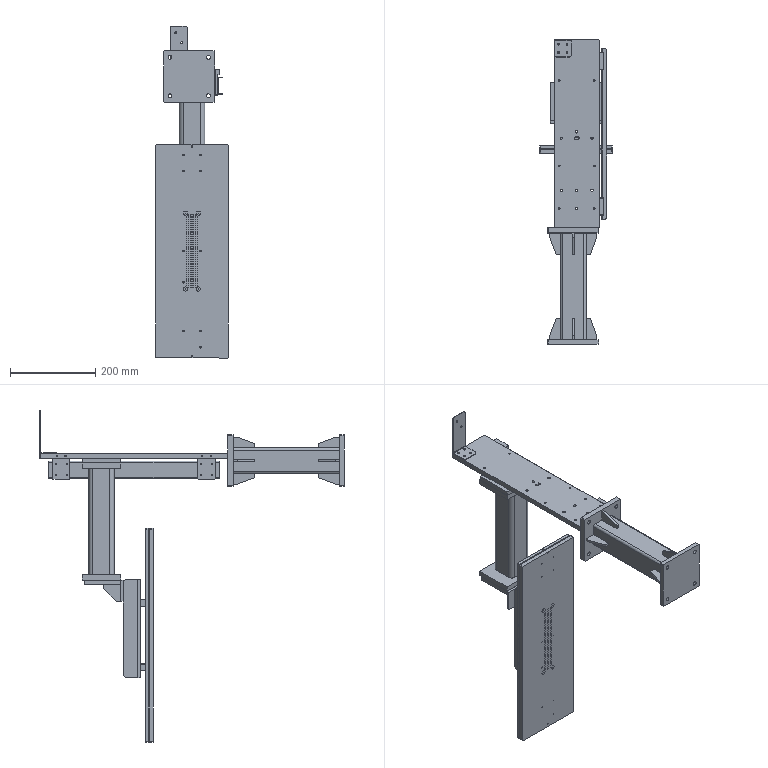Assembly | SolidWorks | mm | 18 component files | 28 solids | 1241 faces | box 170 x 712 x 777.07 mm | volume 4280144 mm3 | cylinder 823 | plane 322 | cone 96 | commonest cylinder face diameters 0.6 x482 3.3 x56 4.2 x44 4.5 x40 10 x40 5.5 x40 8 x24 2.5 x20
Bill of materials:
001 | 1 | Q235B | Welded-style frame made of a long channel or I-section member running between two square end plates, with triangular gusset ribs at both ends.
005 | 1 | AL6061 | Long, thin rectangular plate with a scattered pattern of small holes and one slot on the main face, plus small holes in the narrow edge faces.
006 | 1 | AL6061 | Thick rectangular plate with a grid of round through holes in several sizes and one obround slot.
007 | 1 | AL6061 | Plain solid rectangular plate or block with no visible holes or cutouts.
008 | 1 | AL6061 | Thin rectangular plate with two large round through holes, each flanked by two small holes, plus small holes along the long edges.
009 | 2 | AL6061 | Long rectangular bar with chamfered corners along one long edge at both ends and three small holes in one narrow face.
011 | 2 | AL6061 | Rectangular block with three large round through holes in a row through its main face.
012 | 1 | AL6061 | Thin rectangular sheet or panel with small holes along both long edges and larger holes on the centerline near each end.
013 | 1 | AL6061 | Thin rectangular sheet or panel with a faint dotted pattern in a narrow vertical region near the center of one face.
015 | 1 | SUS304 | Bent L-shaped bracket made of plate with rounded outer corners, holes in both legs.
017 | 1 | SUS304 | Long formed C-channel (U-profile) with rounded bends and groups of small holes near each end of the web.
021 | 1 | AL6061 | Plain thin rectangular plate with no visible holes.
022 | 1 | AL6061 | Solid block shaped like a corner gusset with a constant thickness. Its side profile has a full-width straight top edge, a full-height vertical back edge, a short vertical edge at the outer end, and a long diagonal edge running down to a narrow flat bottom. There are two round holes in the top face and two in the vertical back face.
023 | 1 |  | Column shaped like an I-beam: two flat rectangular end plates of the same size joined by a central rectangular post. The post is narrower than the plates and has rounded vertical edges.
X003.02-011(1)-014 | 2 | AL6061 | Rectangular plate with a thicker stepped lip along one edge, so its side profile is L-shaped. It has two larger round through-holes near the lip edge and four smaller round through-holes in a rectangular pattern lower on the plate. The plate corners are very slightly rounded or chamfered.
Mates:
1. parallel | 006-1 face at (-180.455, -15.942, 144.696) dir (0, 1, 0) | 007-1 face at (-180.455, -21.942, -139.304) dir (0, 1, 0)
2. concentric | 008-2 face at (-275.455, -151.942, -338.376) dir (0, -1, 0) r 2.75 | 009-2 face at (-275.455, -145.942, -338.376) dir (0, -1, 0) r 2.1
3. concentric | 008-2 face at (-275.455, -151.942, -243.376) dir (0, -1, 0) r 2.75 | 009-2 face at (-275.455, -145.942, -243.376) dir (0, -1, 0) r 2.1
4. coincident | 008-2 face at (-240.455, -145.942, -238.376) dir (0, 1, 0) | 009-2 face at (-270.455, -145.942, -358.376) dir (0, -1, 0)
5. concentric | 008-2 face at (-205.455, -151.942, -338.376) dir (0, -1, 0) r 2.75 | 009-1 face at (-205.455, -145.942, -338.376) dir (0, -1, 0) r 2.1
6. concentric | 008-2 face at (-205.455, -151.942, -243.376) dir (0, -1, 0) r 2.75 | 009-1 face at (-205.455, -145.942, -243.376) dir (0, -1, 0) r 2.1
7. coincident | 008-2 face at (-240.455, -145.942, -238.376) dir (0, 1, 0) | 009-1 face at (-200.455, -145.942, -358.376) dir (0, -1, 0)
8. concentric | 011-1 face at (-228.955, -151.942, -183.376) dir (0, 1, 0) r 5 | 012-1 face at (-228.955, -163.942, -183.376) dir (0, 1, 0) r 2.1
9. coincident | 011-1 face at (-240.455, -163.942, -183.376) dir (0, -1, 0) | 012-1 face at (-240.455, -163.942, -258.376) dir (0, 1, 0)
10. concentric | 011-1 face at (-251.955, -151.942, -183.376) dir (0, 1, 0) r 5 | 012-1 face at (-251.955, -163.942, -183.376) dir (0, 1, 0) r 2.1
11. coincident | 011-2 face at (-240.455, -163.942, -333.376) dir (0, -1, 0) | 012-1 face at (-240.455, -163.942, -258.376) dir (0, 1, 0)
12. concentric | 011-2 face at (-228.955, -151.942, -333.376) dir (0, 1, 0) r 5 | 012-1 face at (-228.955, -163.942, -333.376) dir (0, 1, 0) r 2.1
13. concentric | 011-2 face at (-251.955, -151.942, -333.376) dir (0, 1, 0) r 2.75 | 012-1 face at (-251.955, -163.942, -333.376) dir (0, 1, 0) r 2.1
14. coincident | 012-1 face at (-240.455, -171.942, -258.376) dir (0, -1, 0) | 013-1 face at (-240.455, -171.942, -258.376) dir (0, 1, 0)
15. coincident | 012-1 face at (-325.455, -171.942, -8.376) dir (-1, 0, 0) | 013-1 face at (-325.455, -181.942, -8.376) dir (-1, 0, 0)
16. coincident | 012-1 face at (-325.455, -171.942, -508.376) dir (0, 0, -1) | 013-1 face at (-325.455, -181.942, -508.376) dir (0, 0, -1)
17. coincident | X003.02-011(1)-014-2 face at (-186.455, -306.942, 136.696) dir (-1, 0, 0) | 005-1 face at (-186.455, -356.942, 154.696) dir (1, 0, 0)
18. concentric | X003.02-011(1)-014-2 face at (-186.455, -316.942, 160.696) dir (-1, 0, 0) r 2.25 | 005-1 face at (-186.455, -316.942, 160.696) dir (1, 0, 0) r 1.65
19. concentric | X003.02-011(1)-014-2 face at (-186.455, -296.942, 160.696) dir (-1, 0, 0) r 2.25 | 005-1 face at (-186.455, -296.942, 160.696) dir (1, 0, 0) r 1.65
20. coincident | 005-1 face at (-238.955, -136.942, 166.696) dir (0, 0, 1) | 015-1 face at (-271.455, 63.058, 166.696) dir (0, 0, -1)
21. concentric | 005-1 face at (-261.455, 53.058, 166.696) dir (0, 0, 1) r 1.65 | 015-1 face at (-261.455, 53.058, 166.696) dir (0, 0, 1) r 2.25
22. coincident | 005-1 face at (-186.455, 83.058, 154.696) dir (0, 1, 0) | 015-1 face at (-271.455, 83.058, 168.196) dir (0, 1, 0)
23. coincident | 021-1 face at (-240.455, -105.942, -154.304) dir (0, 1, 0) | 022-1 face at (-235.455, -105.942, -139.304) dir (0, -1, 0)
24. coincident | 009-2 face at (-270.455, -111.942, -128.376) dir (0, 1, 0) | 021-1 face at (-240.455, -111.942, -154.304) dir (0, -1, 0)
25. coincident | 006-1 face at (-240.455, -60.942, 144.696) dir (0, 0, -1) | 023-1 face at (-240.455, -60.942, 144.696) dir (0, 0, 1)
26. coincident | 006-1 face at (-180.455, -105.942, 144.696) dir (0, -1, 0) | 023-1 face at (-300.455, -105.942, 132.696) dir (0, -1, 0)
27. width | 023-1 face at (-300.455, -15.942, 132.696) dir (-1, 0, 0) | 023-1 face at (-180.455, -15.942, 132.696) dir (1, 0, 0) | 006-1 face at (-300.455, -105.942, 144.696) dir (-1, 0, 0) | 006-1 face at (-180.455, -105.942, 144.696) dir (1, 0, 0)
28. coincident | X003.02-011(1)-014-2 face at (-180.455, -306.942, 136.696) dir (1, 0, 0) | 017-1 face at (-180.455, -136.942, 129.196) dir (-1, 0, 0)
29. coincident | X003.02-011(1)-014-1 face at (-186.455, 33.058, 136.696) dir (-1, 0, 0) | 005-1 face at (-186.455, -356.942, 154.696) dir (1, 0, 0)
30. concentric | X003.02-011(1)-014-1 face at (-186.455, 43.058, 160.696) dir (-1, 0, 0) r 2.25 | 005-1 face at (-186.455, 43.058, 160.696) dir (1, 0, 0) r 1.65
31. concentric | X003.02-011(1)-014-1 face at (-186.455, 23.058, 160.696) dir (-1, 0, 0) r 2.25 | 005-1 face at (-186.455, 23.058, 160.696) dir (1, 0, 0) r 1.65
32. concentric | X003.02-011(1)-014-1 edge at (-180.455, 45.558, 141.696) dir (1, 0, 0) r 1.25 | 017-1 edge at (-178.955, 45.558, 141.696) dir (1, 0, 0) r 3.3
33. concentric | X003.02-011(1)-014-2 edge at (-180.455, -319.442, 141.696) dir (1, 0, 0) r 1.25 | 017-1 edge at (-178.955, -319.442, 141.696) dir (1, 0, 0) r 3.3
34. width | 021-1 face at (-180.455, -111.942, -129.304) dir (1, 0, 0) | 021-1 face at (-300.455, -111.942, -129.304) dir (-1, 0, 0) | 009-2 face at (-280.455, -145.942, -128.376) dir (-1, 0, 0) | 009-1 face at (-200.455, -145.942, -128.376) dir (1, 0, 0)
35. coincident | 007-1 face at (-180.455, -105.942, -139.304) dir (0, -1, 0) | 021-1 face at (-240.455, -105.942, -154.304) dir (0, 1, 0)
36. coincident | 007-1 face at (-180.455, -105.942, -139.304) dir (1, 0, 0) | 021-1 face at (-180.455, -111.942, -129.304) dir (1, 0, 0)
37. coincident | 007-1 face at (-240.455, -63.942, -129.304) dir (0, 0, 1) | 021-1 face at (-300.455, -111.942, -129.304) dir (0, 0, 1)
38. coincident | 007-1 face at (-240.455, -63.942, -129.304) dir (0, 0, 1) | 023-1 face at (-240.455, -60.942, -129.304) dir (0, 0, -1)
39. coincident | 007-1 face at (-240.455, -63.942, -139.304) dir (0, 0, -1) | 022-1 face at (-235.455, -105.942, -139.304) dir (0, 0, 1)
40. width | 007-1 face at (-180.455, -105.942, -139.304) dir (1, 0, 0) | 007-1 face at (-300.455, -105.942, -139.304) dir (-1, 0, 0) | 023-1 face at (-300.455, -105.942, -129.304) dir (-1, 0, 0) | 023-1 face at (-180.455, -15.942, -129.304) dir (1, 0, 0)
41. coincident | 021-1 face at (-240.455, -105.942, -154.304) dir (0, 1, 0) | 023-1 face at (-180.455, -105.942, -129.304) dir (0, -1, 0)
42. width | 022-1 face at (-235.455, -85.942, -159.304) dir (1, 0, 0) | 022-1 face at (-245.455, -85.942, -159.304) dir (-1, 0, 0) | 007-1 face at (-300.455, -105.942, -139.304) dir (-1, 0, 0) | 007-1 face at (-180.455, -105.942, -139.304) dir (1, 0, 0)
43. coincident | 005-1 face at (-238.955, -136.942, 154.696) dir (0, 0, -1) | 006-1 face at (-240.455, -60.942, 154.696) dir (0, 0, 1)
44. concentric | 008-2 face at (-240.455, -145.942, -183.376) dir (0, -1, 0) r 9.5 | 011-1 face at (-240.455, -163.942, -183.376) dir (0, -1, 0) r 2.75
45. coincident | 017-1 face at (-180.455, -136.942, 129.196) dir (-1, 0, 0) | 023-1 face at (-180.455, -15.942, 132.696) dir (1, 0, 0)